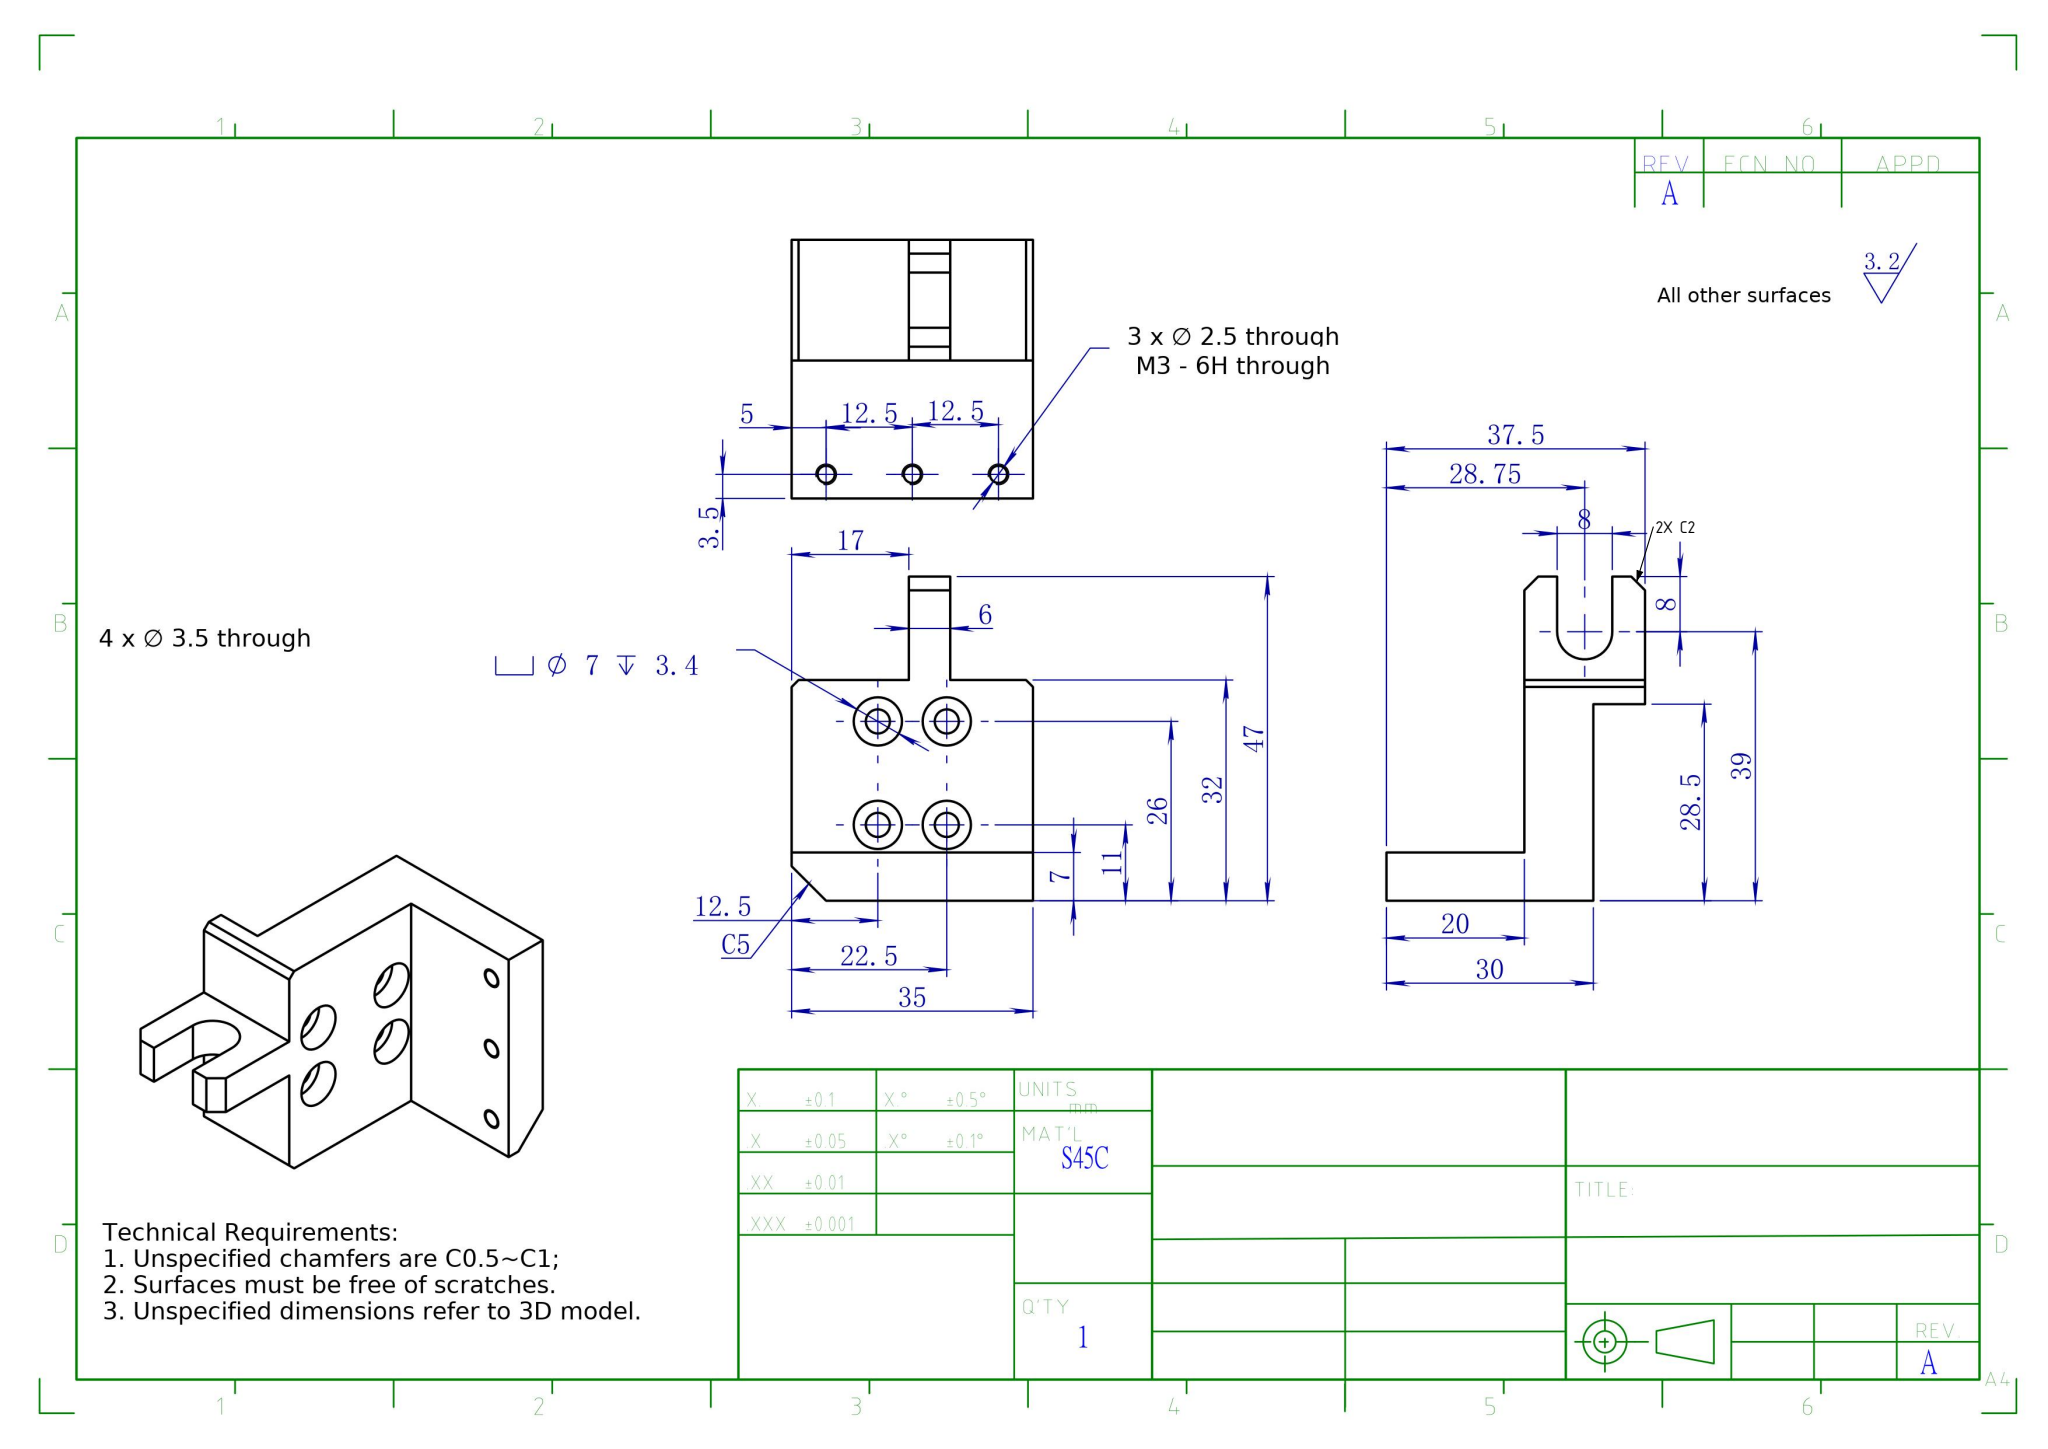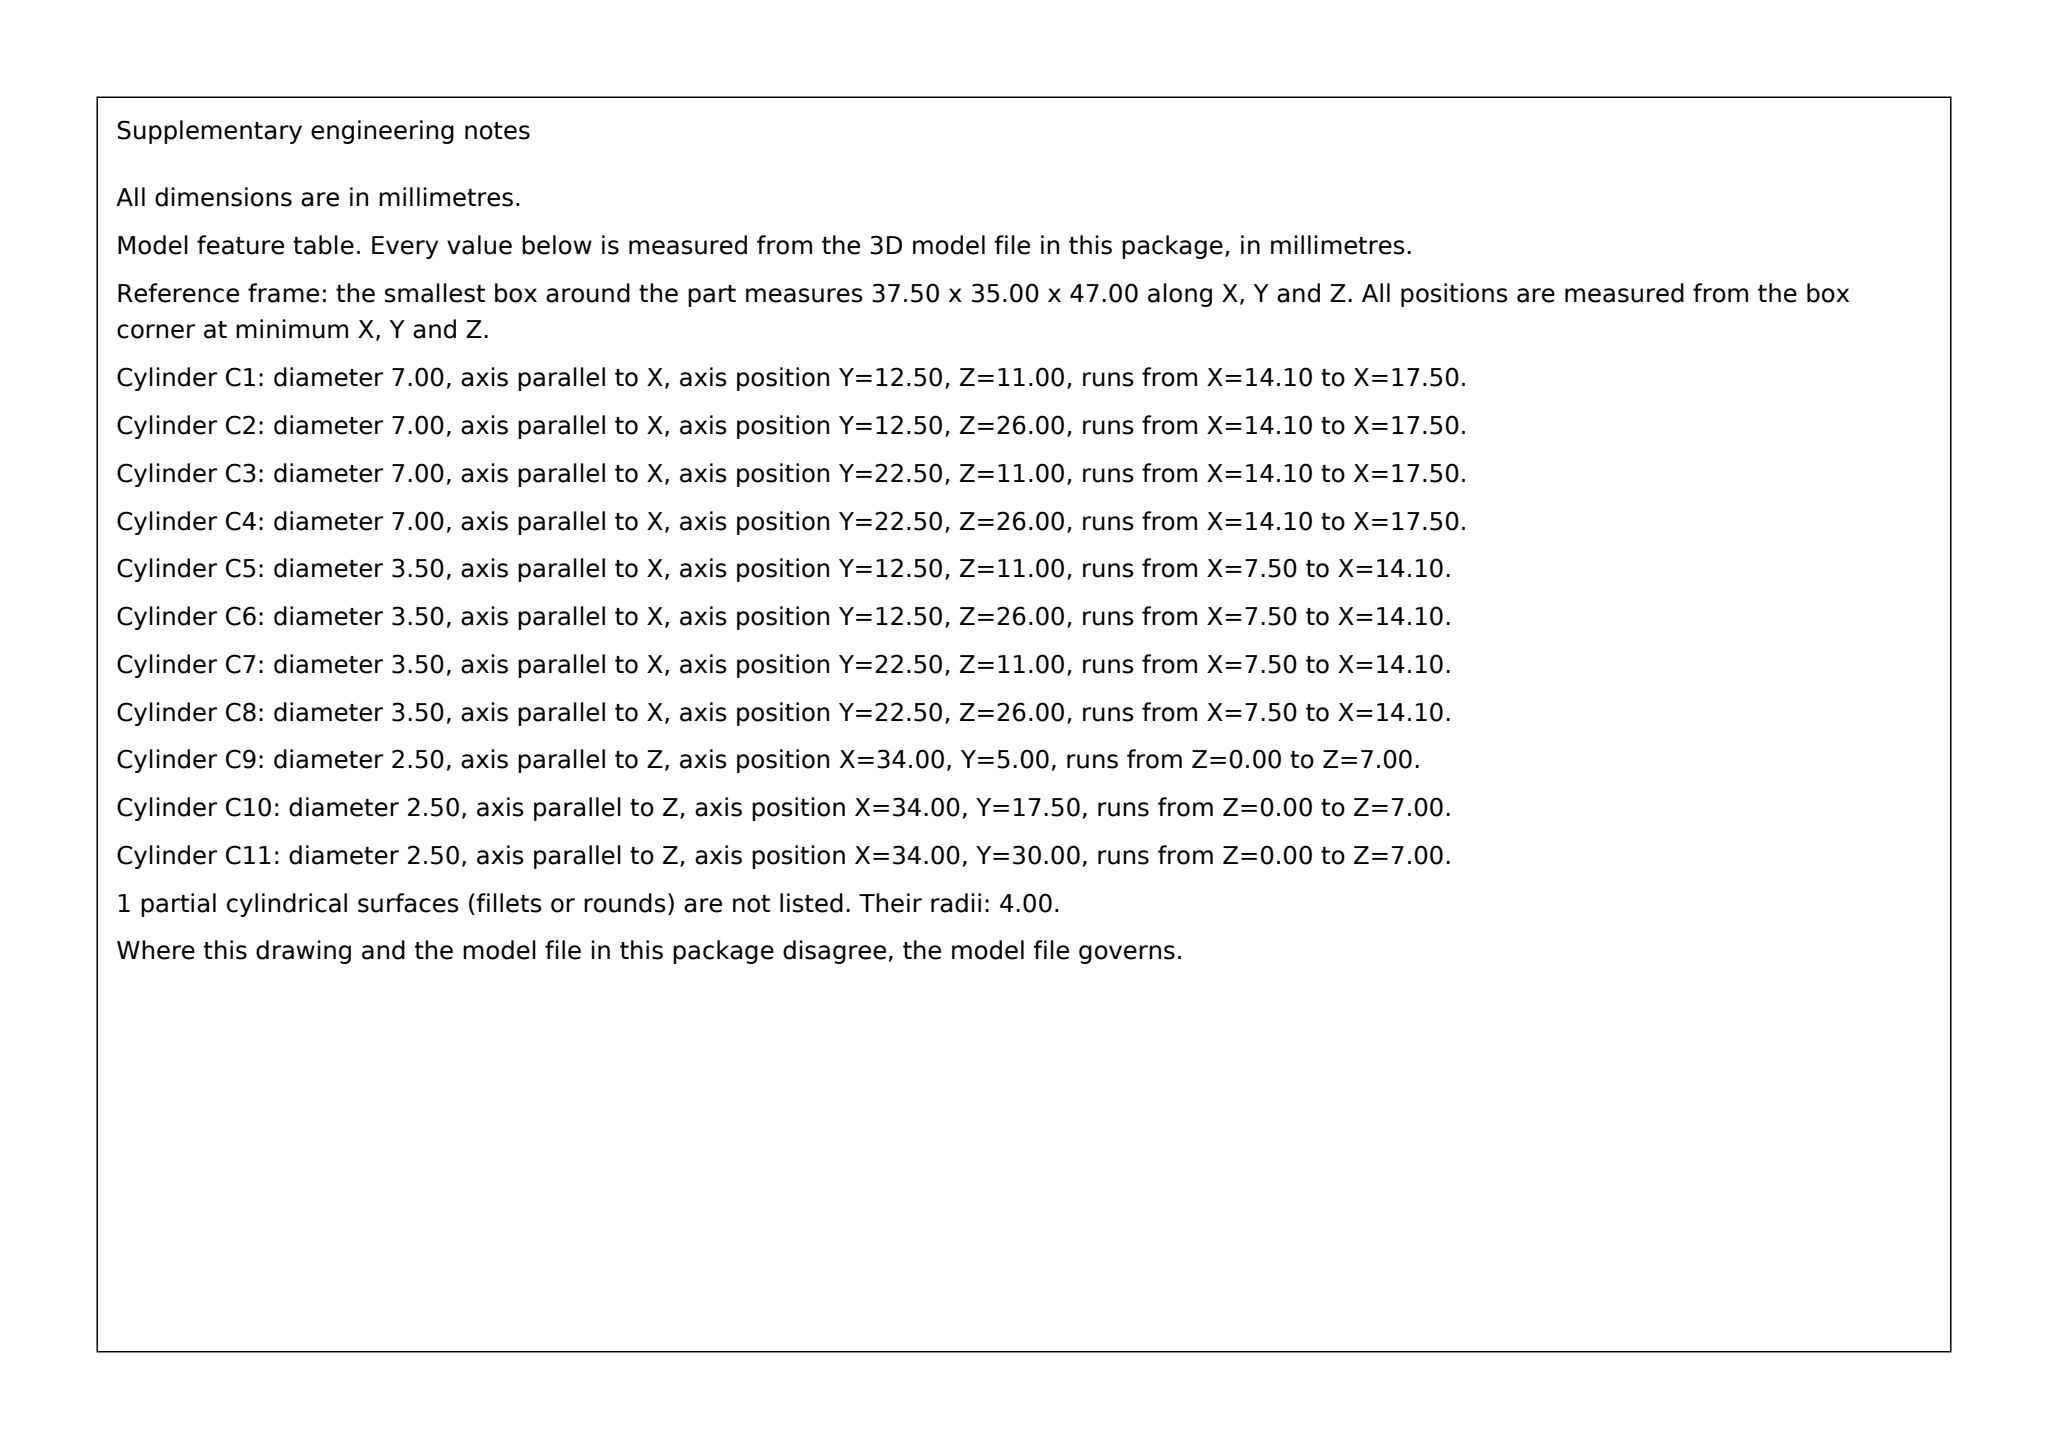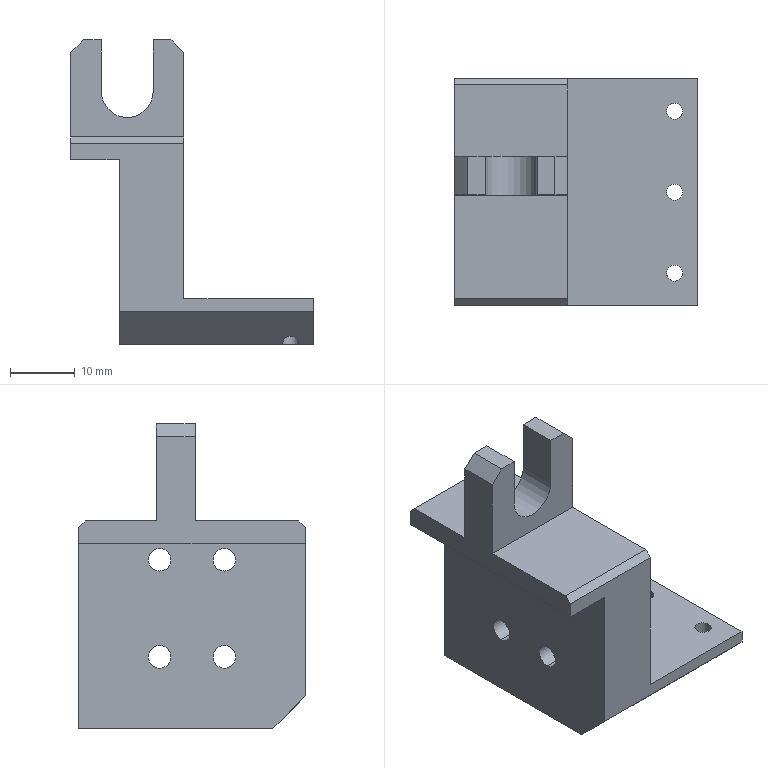Part | SolidWorks | mm | material S45C | 1 solid | 49 faces | box 37.5 x 35 x 47 mm | volume 16763 mm3 | plane 26 | cylinder 23 | commonest cylinder face diameters 7 x8 3.5 x8 2.5 x6 8 x1
Drawing notes:
2X CHAMFER 2 x 45° ON TOP OUTER CORNERS OF FORK PRONGS: from top face (47 from base) down 2, and 2 in from each outer prong face (X 0 and X 17.5); chamfer runs full 6 prong width. | from the solid: inclined_planes: angle_to_xyz_axes [45.0,90.0,45.0] at bbox_from [0.0,17.0,45.0] size [2,6,2] and bbox_from [15.5,17.0,45.0] size [2,6,2]